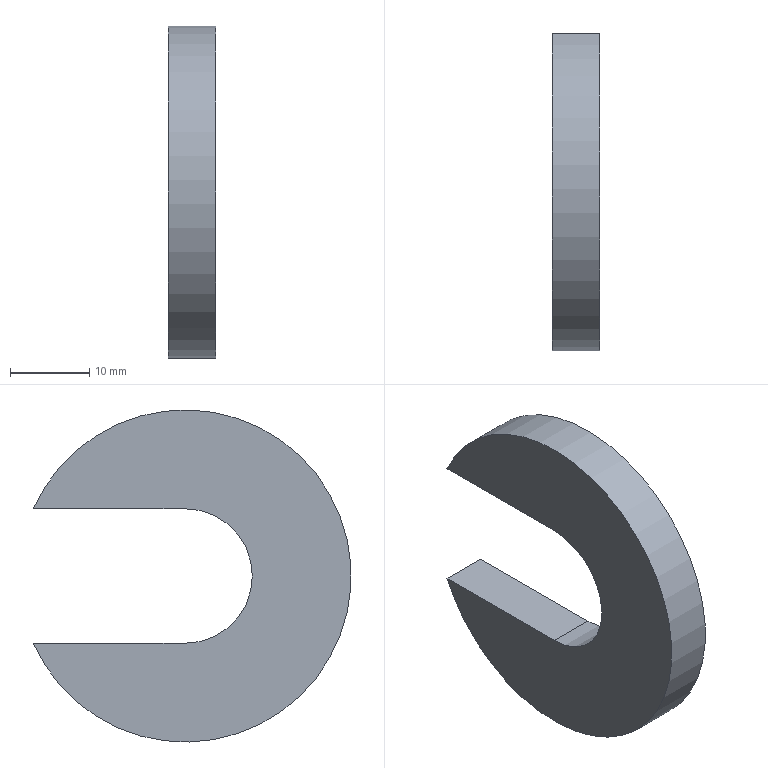Component | NX | 36_PAD_BLOCK | 1 solid | 6 faces | box 6 x 40.2 x 42 mm | volume 5550 mm3 | plane 4 | cylinder 2 | commonest cylinder face diameters 17 x1 42 x1
STEP:
#1=CARTESIAN_POINT('',(0.,0.,0.));
#2=DIRECTION('',(0.,0.,1.));
#3=DIRECTION('',(1.,0.,0.));
#4=AXIS2_PLACEMENT_3D('',#1,#2,#3);
#5=CARTESIAN_POINT('',(56.,40.,-8.5));
#6=VERTEX_POINT('',#5);
#7=CARTESIAN_POINT('',(50.,40.,-8.5));
#8=VERTEX_POINT('',#7);
#9=CARTESIAN_POINT('',(56.,40.,-8.5));
#10=DIRECTION('',(-1.,0.,0.));
#11=VECTOR('',#10,1.);
#12=LINE('',#9,#11);
#13=CARTESIAN_POINT('',(56.,40.,-0.));
#14=DIRECTION('',(-1.,0.,0.));
#15=DIRECTION('',(0.,-1.,0.));
#16=AXIS2_PLACEMENT_3D('',#13,#14,#15);
#17=CYLINDRICAL_SURFACE('',#16,8.5);
#18=CARTESIAN_POINT('',(4.712,0.));
#19=DIRECTION('',(0.,1.));
#20=VECTOR('',#19,1.);
#21=LINE('',#18,#20);
#22=(GEOMETRIC_REPRESENTATION_CONTEXT(2)PARAMETRIC_REPRESENTATION_CONTEXT()REPRESENTATION_CONTEXT('',''));
#23=DEFINITIONAL_REPRESENTATION('',(#21),#22);
#24=PCURVE('',#17,#23);
#25=CARTESIAN_POINT('',(56.,59.203,-8.5));
#26=DIRECTION('',(0.,0.,-1.));
#27=DIRECTION('',(-1.,0.,0.));
#28=AXIS2_PLACEMENT_3D('',#25,#26,#27);
#29=PLANE('',#28);
#30=CARTESIAN_POINT('',(0.,-19.203));
#31=DIRECTION('',(1.,0.));
#32=VECTOR('',#31,1.);
#33=LINE('',#30,#32);
#34=(GEOMETRIC_REPRESENTATION_CONTEXT(2)PARAMETRIC_REPRESENTATION_CONTEXT()REPRESENTATION_CONTEXT('',''));
#35=DEFINITIONAL_REPRESENTATION('',(#33),#34);
#36=PCURVE('',#29,#35);
#37=SURFACE_CURVE('',#12,(#24,#36),.PCURVE_S1.);
#38=EDGE_CURVE('',#6,#8,#37,.T.);
#39=ORIENTED_EDGE('',*,*,#38,.F.);
#40=CARTESIAN_POINT('',(56.,40.,8.5));
#41=VERTEX_POINT('',#40);
#42=CARTESIAN_POINT('',(56.,40.,-0.));
#43=DIRECTION('',(-1.,0.,0.));
#44=DIRECTION('',(0.,1.,0.));
#45=AXIS2_PLACEMENT_3D('',#42,#43,#44);
#46=CIRCLE('',#45,8.5);
#47=CARTESIAN_POINT('',(3.142,0.));
#48=DIRECTION('',(1.,0.));
#49=VECTOR('',#48,1.);
#50=LINE('',#47,#49);
#51=(GEOMETRIC_REPRESENTATION_CONTEXT(2)PARAMETRIC_REPRESENTATION_CONTEXT()REPRESENTATION_CONTEXT('',''));
#52=DEFINITIONAL_REPRESENTATION('',(#50),#51);
#53=PCURVE('',#17,#52);
#54=CARTESIAN_POINT('',(56.,40.,-0.));
#55=DIRECTION('',(-1.,0.,0.));
#56=DIRECTION('',(0.,-1.,0.));
#57=AXIS2_PLACEMENT_3D('',#54,#55,#56);
#58=PLANE('',#57);
#59=CARTESIAN_POINT('',(0.,0.));
#60=DIRECTION('',(-1.,0.));
#61=AXIS2_PLACEMENT_2D('',#59,#60);
#62=CIRCLE('',#61,8.5);
#63=(GEOMETRIC_REPRESENTATION_CONTEXT(2)PARAMETRIC_REPRESENTATION_CONTEXT()REPRESENTATION_CONTEXT('',''));
#64=DEFINITIONAL_REPRESENTATION('',(#62),#63);
#65=PCURVE('',#58,#64);
#66=SURFACE_CURVE('',#46,(#53,#65),.PCURVE_S1.);
#67=EDGE_CURVE('',#6,#41,#66,.T.);
#68=ORIENTED_EDGE('',*,*,#67,.T.);
#69=CARTESIAN_POINT('',(50.,40.,8.5));
#70=VERTEX_POINT('',#69);
#71=CARTESIAN_POINT('',(56.,40.,8.5));
#72=DIRECTION('',(-1.,0.,0.));
#73=VECTOR('',#72,1.);
#74=LINE('',#71,#73);
#75=CARTESIAN_POINT('',(7.854,0.));
#76=DIRECTION('',(0.,1.));
#77=VECTOR('',#76,1.);
#78=LINE('',#75,#77);
#79=(GEOMETRIC_REPRESENTATION_CONTEXT(2)PARAMETRIC_REPRESENTATION_CONTEXT()REPRESENTATION_CONTEXT('',''));
#80=DEFINITIONAL_REPRESENTATION('',(#78),#79);
#81=PCURVE('',#17,#80);
#82=CARTESIAN_POINT('',(56.,40.,8.5));
#83=DIRECTION('',(0.,0.,1.));
#84=DIRECTION('',(1.,0.,0.));
#85=AXIS2_PLACEMENT_3D('',#82,#83,#84);
#86=PLANE('',#85);
#87=CARTESIAN_POINT('',(0.,0.));
#88=DIRECTION('',(-1.,0.));
#89=VECTOR('',#88,1.);
#90=LINE('',#87,#89);
#91=(GEOMETRIC_REPRESENTATION_CONTEXT(2)PARAMETRIC_REPRESENTATION_CONTEXT()REPRESENTATION_CONTEXT('',''));
#92=DEFINITIONAL_REPRESENTATION('',(#90),#91);
#93=PCURVE('',#86,#92);
#94=SURFACE_CURVE('',#74,(#81,#93),.PCURVE_S1.);
#95=EDGE_CURVE('',#41,#70,#94,.T.);
#96=ORIENTED_EDGE('',*,*,#95,.T.);
#97=CARTESIAN_POINT('',(50.,40.,-0.));
#98=DIRECTION('',(-1.,0.,0.));
#99=DIRECTION('',(0.,1.,0.));
#100=AXIS2_PLACEMENT_3D('',#97,#98,#99);
#101=CIRCLE('',#100,8.5);
#102=CARTESIAN_POINT('',(3.142,6.));
#103=DIRECTION('',(1.,0.));
#104=VECTOR('',#103,1.);
#105=LINE('',#102,#104);
#106=(GEOMETRIC_REPRESENTATION_CONTEXT(2)PARAMETRIC_REPRESENTATION_CONTEXT()REPRESENTATION_CONTEXT('',''));
#107=DEFINITIONAL_REPRESENTATION('',(#105),#106);
#108=PCURVE('',#17,#107);
#109=CARTESIAN_POINT('',(50.,40.,-0.));
#110=DIRECTION('',(-1.,0.,0.));
#111=DIRECTION('',(0.,-1.,0.));
#112=AXIS2_PLACEMENT_3D('',#109,#110,#111);
#113=PLANE('',#112);
#114=CARTESIAN_POINT('',(0.,0.));
#115=DIRECTION('',(-1.,0.));
#116=AXIS2_PLACEMENT_2D('',#114,#115);
#117=CIRCLE('',#116,8.5);
#118=(GEOMETRIC_REPRESENTATION_CONTEXT(2)PARAMETRIC_REPRESENTATION_CONTEXT()REPRESENTATION_CONTEXT('',''));
#119=DEFINITIONAL_REPRESENTATION('',(#117),#118);
#120=PCURVE('',#113,#119);
#121=SURFACE_CURVE('',#101,(#108,#120),.PCURVE_S1.);
#122=EDGE_CURVE('',#8,#70,#121,.T.);
#123=ORIENTED_EDGE('',*,*,#122,.F.);
#124=EDGE_LOOP('',(#39,#68,#96,#123));
#125=FACE_BOUND('',#124,.F.);
#126=ADVANCED_FACE('',(#125),#17,.F.);
#127=CARTESIAN_POINT('',(50.,59.203,8.5));
#128=VERTEX_POINT('',#127);
#129=CARTESIAN_POINT('',(50.,40.,8.5));
#130=DIRECTION('',(0.,1.,0.));
#131=VECTOR('',#130,1.);
#132=LINE('',#129,#131);
#133=CARTESIAN_POINT('',(-6.,0.));
#134=DIRECTION('',(0.,1.));
#135=VECTOR('',#134,1.);
#136=LINE('',#133,#135);
#137=(GEOMETRIC_REPRESENTATION_CONTEXT(2)PARAMETRIC_REPRESENTATION_CONTEXT()REPRESENTATION_CONTEXT('',''));
#138=DEFINITIONAL_REPRESENTATION('',(#136),#137);
#139=PCURVE('',#86,#138);
#140=CARTESIAN_POINT('',(0.,8.5));
#141=DIRECTION('',(-1.,0.));
#142=VECTOR('',#141,1.);
#143=LINE('',#140,#142);
#144=(GEOMETRIC_REPRESENTATION_CONTEXT(2)PARAMETRIC_REPRESENTATION_CONTEXT()REPRESENTATION_CONTEXT('',''));
#145=DEFINITIONAL_REPRESENTATION('',(#143),#144);
#146=PCURVE('',#113,#145);
#147=SURFACE_CURVE('',#132,(#139,#146),.PCURVE_S1.);
#148=EDGE_CURVE('',#70,#128,#147,.T.);
#149=ORIENTED_EDGE('',*,*,#148,.T.);
#150=CARTESIAN_POINT('',(56.,59.203,8.5));
#151=VERTEX_POINT('',#150);
#152=CARTESIAN_POINT('',(56.,59.203,8.5));
#153=DIRECTION('',(-1.,0.,0.));
#154=VECTOR('',#153,1.);
#155=LINE('',#152,#154);
#156=CARTESIAN_POINT('',(0.,19.203));
#157=DIRECTION('',(-1.,0.));
#158=VECTOR('',#157,1.);
#159=LINE('',#156,#158);
#160=(GEOMETRIC_REPRESENTATION_CONTEXT(2)PARAMETRIC_REPRESENTATION_CONTEXT()REPRESENTATION_CONTEXT('',''));
#161=DEFINITIONAL_REPRESENTATION('',(#159),#160);
#162=PCURVE('',#86,#161);
#163=CARTESIAN_POINT('',(56.,40.,-0.));
#164=DIRECTION('',(-1.,0.,0.));
#165=DIRECTION('',(0.,-1.,0.));
#166=AXIS2_PLACEMENT_3D('',#163,#164,#165);
#167=CYLINDRICAL_SURFACE('',#166,21.);
#168=CARTESIAN_POINT('',(2.725,0.));
#169=DIRECTION('',(0.,1.));
#170=VECTOR('',#169,1.);
#171=LINE('',#168,#170);
#172=(GEOMETRIC_REPRESENTATION_CONTEXT(2)PARAMETRIC_REPRESENTATION_CONTEXT()REPRESENTATION_CONTEXT('',''));
#173=DEFINITIONAL_REPRESENTATION('',(#171),#172);
#174=PCURVE('',#167,#173);
#175=SURFACE_CURVE('',#155,(#162,#174),.PCURVE_S1.);
#176=EDGE_CURVE('',#151,#128,#175,.T.);
#177=ORIENTED_EDGE('',*,*,#176,.F.);
#178=CARTESIAN_POINT('',(56.,40.,8.5));
#179=DIRECTION('',(0.,1.,0.));
#180=VECTOR('',#179,1.);
#181=LINE('',#178,#180);
#182=CARTESIAN_POINT('',(0.,0.));
#183=DIRECTION('',(0.,1.));
#184=VECTOR('',#183,1.);
#185=LINE('',#182,#184);
#186=(GEOMETRIC_REPRESENTATION_CONTEXT(2)PARAMETRIC_REPRESENTATION_CONTEXT()REPRESENTATION_CONTEXT('',''));
#187=DEFINITIONAL_REPRESENTATION('',(#185),#186);
#188=PCURVE('',#86,#187);
#189=CARTESIAN_POINT('',(0.,8.5));
#190=DIRECTION('',(-1.,0.));
#191=VECTOR('',#190,1.);
#192=LINE('',#189,#191);
#193=(GEOMETRIC_REPRESENTATION_CONTEXT(2)PARAMETRIC_REPRESENTATION_CONTEXT()REPRESENTATION_CONTEXT('',''));
#194=DEFINITIONAL_REPRESENTATION('',(#192),#193);
#195=PCURVE('',#58,#194);
#196=SURFACE_CURVE('',#181,(#188,#195),.PCURVE_S1.);
#197=EDGE_CURVE('',#41,#151,#196,.T.);
#198=ORIENTED_EDGE('',*,*,#197,.F.);
#199=ORIENTED_EDGE('',*,*,#95,.T.);
#200=EDGE_LOOP('',(#149,#177,#198,#199));
#201=FACE_BOUND('',#200,.T.);
#202=ADVANCED_FACE('',(#201),#86,.F.);
#203=CARTESIAN_POINT('',(50.,59.203,-8.5));
#204=VERTEX_POINT('',#203);
#205=CARTESIAN_POINT('',(50.,40.,-0.));
#206=DIRECTION('',(1.,0.,0.));
#207=DIRECTION('',(0.,1.,0.));
#208=AXIS2_PLACEMENT_3D('',#205,#206,#207);
#209=CIRCLE('',#208,21.);
#210=CARTESIAN_POINT('',(3.142,6.));
#211=DIRECTION('',(-1.,0.));
#212=VECTOR('',#211,1.);
#213=LINE('',#210,#212);
#214=(GEOMETRIC_REPRESENTATION_CONTEXT(2)PARAMETRIC_REPRESENTATION_CONTEXT()REPRESENTATION_CONTEXT('',''));
#215=DEFINITIONAL_REPRESENTATION('',(#213),#214);
#216=PCURVE('',#167,#215);
#217=CARTESIAN_POINT('',(-21.,0.));
#218=CARTESIAN_POINT('',(-21.,36.373));
#219=CARTESIAN_POINT('',(10.5,18.187));
#220=CARTESIAN_POINT('',(42.,0.));
#221=CARTESIAN_POINT('',(10.5,-18.187));
#222=CARTESIAN_POINT('',(-21.,-36.373));
#223=CARTESIAN_POINT('',(-21.,0.));
#224=(BOUNDED_CURVE()B_SPLINE_CURVE(2,(#217,#218,#219,#220,#221,#222,#223),.UNSPECIFIED.,.T.,.F.)B_SPLINE_CURVE_WITH_KNOTS((1,2,2,2,2,1),(-2.094,0.,2.094,4.189,6.283,8.378),.UNSPECIFIED.)CURVE()GEOMETRIC_REPRESENTATION_ITEM()RATIONAL_B_SPLINE_CURVE((1.,0.5,1.,0.5,1.,0.5,1.))REPRESENTATION_ITEM(''));
#225=(GEOMETRIC_REPRESENTATION_CONTEXT(2)PARAMETRIC_REPRESENTATION_CONTEXT()REPRESENTATION_CONTEXT('',''));
#226=DEFINITIONAL_REPRESENTATION('',(#224),#225);
#227=PCURVE('',#113,#226);
#228=SURFACE_CURVE('',#209,(#216,#227),.PCURVE_S1.);
#229=EDGE_CURVE('',#128,#204,#228,.T.);
#230=ORIENTED_EDGE('',*,*,#229,.T.);
#231=CARTESIAN_POINT('',(56.,59.203,-8.5));
#232=VERTEX_POINT('',#231);
#233=CARTESIAN_POINT('',(56.,59.203,-8.5));
#234=DIRECTION('',(-1.,0.,0.));
#235=VECTOR('',#234,1.);
#236=LINE('',#233,#235);
#237=CARTESIAN_POINT('',(-2.725,0.));
#238=DIRECTION('',(0.,1.));
#239=VECTOR('',#238,1.);
#240=LINE('',#237,#239);
#241=(GEOMETRIC_REPRESENTATION_CONTEXT(2)PARAMETRIC_REPRESENTATION_CONTEXT()REPRESENTATION_CONTEXT('',''));
#242=DEFINITIONAL_REPRESENTATION('',(#240),#241);
#243=PCURVE('',#167,#242);
#244=CARTESIAN_POINT('',(0.,0.));
#245=DIRECTION('',(1.,0.));
#246=VECTOR('',#245,1.);
#247=LINE('',#244,#246);
#248=(GEOMETRIC_REPRESENTATION_CONTEXT(2)PARAMETRIC_REPRESENTATION_CONTEXT()REPRESENTATION_CONTEXT('',''));
#249=DEFINITIONAL_REPRESENTATION('',(#247),#248);
#250=PCURVE('',#29,#249);
#251=SURFACE_CURVE('',#236,(#243,#250),.PCURVE_S1.);
#252=EDGE_CURVE('',#232,#204,#251,.T.);
#253=ORIENTED_EDGE('',*,*,#252,.F.);
#254=CARTESIAN_POINT('',(56.,40.,-0.));
#255=DIRECTION('',(1.,0.,0.));
#256=DIRECTION('',(0.,1.,0.));
#257=AXIS2_PLACEMENT_3D('',#254,#255,#256);
#258=CIRCLE('',#257,21.);
#259=CARTESIAN_POINT('',(3.142,0.));
#260=DIRECTION('',(-1.,0.));
#261=VECTOR('',#260,1.);
#262=LINE('',#259,#261);
#263=(GEOMETRIC_REPRESENTATION_CONTEXT(2)PARAMETRIC_REPRESENTATION_CONTEXT()REPRESENTATION_CONTEXT('',''));
#264=DEFINITIONAL_REPRESENTATION('',(#262),#263);
#265=PCURVE('',#167,#264);
#266=CARTESIAN_POINT('',(-21.,0.));
#267=CARTESIAN_POINT('',(-21.,36.373));
#268=CARTESIAN_POINT('',(10.5,18.187));
#269=CARTESIAN_POINT('',(42.,0.));
#270=CARTESIAN_POINT('',(10.5,-18.187));
#271=CARTESIAN_POINT('',(-21.,-36.373));
#272=CARTESIAN_POINT('',(-21.,0.));
#273=(BOUNDED_CURVE()B_SPLINE_CURVE(2,(#266,#267,#268,#269,#270,#271,#272),.UNSPECIFIED.,.T.,.F.)B_SPLINE_CURVE_WITH_KNOTS((1,2,2,2,2,1),(-2.094,0.,2.094,4.189,6.283,8.378),.UNSPECIFIED.)CURVE()GEOMETRIC_REPRESENTATION_ITEM()RATIONAL_B_SPLINE_CURVE((1.,0.5,1.,0.5,1.,0.5,1.))REPRESENTATION_ITEM(''));
#274=(GEOMETRIC_REPRESENTATION_CONTEXT(2)PARAMETRIC_REPRESENTATION_CONTEXT()REPRESENTATION_CONTEXT('',''));
#275=DEFINITIONAL_REPRESENTATION('',(#273),#274);
#276=PCURVE('',#58,#275);
#277=SURFACE_CURVE('',#258,(#265,#276),.PCURVE_S1.);
#278=EDGE_CURVE('',#151,#232,#277,.T.);
#279=ORIENTED_EDGE('',*,*,#278,.F.);
#280=ORIENTED_EDGE('',*,*,#176,.T.);
#281=EDGE_LOOP('',(#230,#253,#279,#280));
#282=FACE_BOUND('',#281,.T.);
#283=ADVANCED_FACE('',(#282),#167,.T.);
#284=CARTESIAN_POINT('',(50.,59.203,-8.5));
#285=DIRECTION('',(0.,-1.,0.));
#286=VECTOR('',#285,1.);
#287=LINE('',#284,#286);
#288=CARTESIAN_POINT('',(6.,0.));
#289=DIRECTION('',(0.,-1.));
#290=VECTOR('',#289,1.);
#291=LINE('',#288,#290);
#292=(GEOMETRIC_REPRESENTATION_CONTEXT(2)PARAMETRIC_REPRESENTATION_CONTEXT()REPRESENTATION_CONTEXT('',''));
#293=DEFINITIONAL_REPRESENTATION('',(#291),#292);
#294=PCURVE('',#29,#293);
#295=CARTESIAN_POINT('',(-19.203,-8.5));
#296=DIRECTION('',(1.,0.));
#297=VECTOR('',#296,1.);
#298=LINE('',#295,#297);
#299=(GEOMETRIC_REPRESENTATION_CONTEXT(2)PARAMETRIC_REPRESENTATION_CONTEXT()REPRESENTATION_CONTEXT('',''));
#300=DEFINITIONAL_REPRESENTATION('',(#298),#299);
#301=PCURVE('',#113,#300);
#302=SURFACE_CURVE('',#287,(#294,#301),.PCURVE_S1.);
#303=EDGE_CURVE('',#204,#8,#302,.T.);
#304=ORIENTED_EDGE('',*,*,#303,.T.);
#305=ORIENTED_EDGE('',*,*,#38,.F.);
#306=CARTESIAN_POINT('',(56.,59.203,-8.5));
#307=DIRECTION('',(0.,-1.,0.));
#308=VECTOR('',#307,1.);
#309=LINE('',#306,#308);
#310=CARTESIAN_POINT('',(0.,0.));
#311=DIRECTION('',(0.,-1.));
#312=VECTOR('',#311,1.);
#313=LINE('',#310,#312);
#314=(GEOMETRIC_REPRESENTATION_CONTEXT(2)PARAMETRIC_REPRESENTATION_CONTEXT()REPRESENTATION_CONTEXT('',''));
#315=DEFINITIONAL_REPRESENTATION('',(#313),#314);
#316=PCURVE('',#29,#315);
#317=CARTESIAN_POINT('',(-19.203,-8.5));
#318=DIRECTION('',(1.,0.));
#319=VECTOR('',#318,1.);
#320=LINE('',#317,#319);
#321=(GEOMETRIC_REPRESENTATION_CONTEXT(2)PARAMETRIC_REPRESENTATION_CONTEXT()REPRESENTATION_CONTEXT('',''));
#322=DEFINITIONAL_REPRESENTATION('',(#320),#321);
#323=PCURVE('',#58,#322);
#324=SURFACE_CURVE('',#309,(#316,#323),.PCURVE_S1.);
#325=EDGE_CURVE('',#232,#6,#324,.T.);
#326=ORIENTED_EDGE('',*,*,#325,.F.);
#327=ORIENTED_EDGE('',*,*,#252,.T.);
#328=EDGE_LOOP('',(#304,#305,#326,#327));
#329=FACE_BOUND('',#328,.T.);
#330=ADVANCED_FACE('',(#329),#29,.F.);
#331=ORIENTED_EDGE('',*,*,#67,.T.);
#332=ORIENTED_EDGE('',*,*,#197,.T.);
#333=ORIENTED_EDGE('',*,*,#278,.T.);
#334=ORIENTED_EDGE('',*,*,#325,.T.);
#335=EDGE_LOOP('',(#331,#332,#333,#334));
#336=FACE_BOUND('',#335,.T.);
#337=ADVANCED_FACE('',(#336),#58,.F.);
#338=ORIENTED_EDGE('',*,*,#122,.F.);
#339=ORIENTED_EDGE('',*,*,#303,.F.);
#340=ORIENTED_EDGE('',*,*,#229,.F.);
#341=ORIENTED_EDGE('',*,*,#148,.F.);
#342=EDGE_LOOP('',(#338,#339,#340,#341));
#343=FACE_BOUND('',#342,.T.);
#344=ADVANCED_FACE('',(#343),#113,.T.);
#345=CLOSED_SHELL('',(#126,#202,#283,#330,#337,#344));
#346=MANIFOLD_SOLID_BREP('',#345);
#347=(LENGTH_UNIT()NAMED_UNIT(*)SI_UNIT(.MILLI.,.METRE.));
#348=UNCERTAINTY_MEASURE_WITH_UNIT(LENGTH_MEASURE(0.0000001),#347,'','');
#349=(NAMED_UNIT(*)PLANE_ANGLE_UNIT()SI_UNIT($,.RADIAN.));
#350=(NAMED_UNIT(*)SI_UNIT($,.STERADIAN.)SOLID_ANGLE_UNIT());
#351=(GEOMETRIC_REPRESENTATION_CONTEXT(3)GLOBAL_UNCERTAINTY_ASSIGNED_CONTEXT((#348))GLOBAL_UNIT_ASSIGNED_CONTEXT((#347,#349,#350))REPRESENTATION_CONTEXT('',''));
#352=ADVANCED_BREP_SHAPE_REPRESENTATION('',(#4,#346),#351);